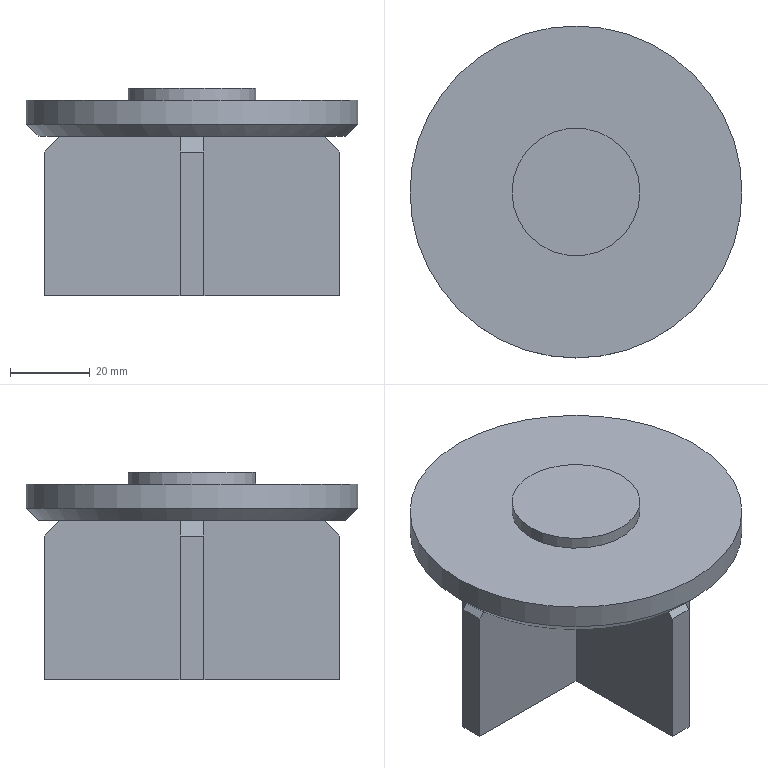Component | NX | 05__VALVE__2 | 1 solid | 23 faces | volume 83851 mm3 | plane 20 | cylinder 2 | cone 1 | commonest cylinder face diameters 83 x1 32 x1